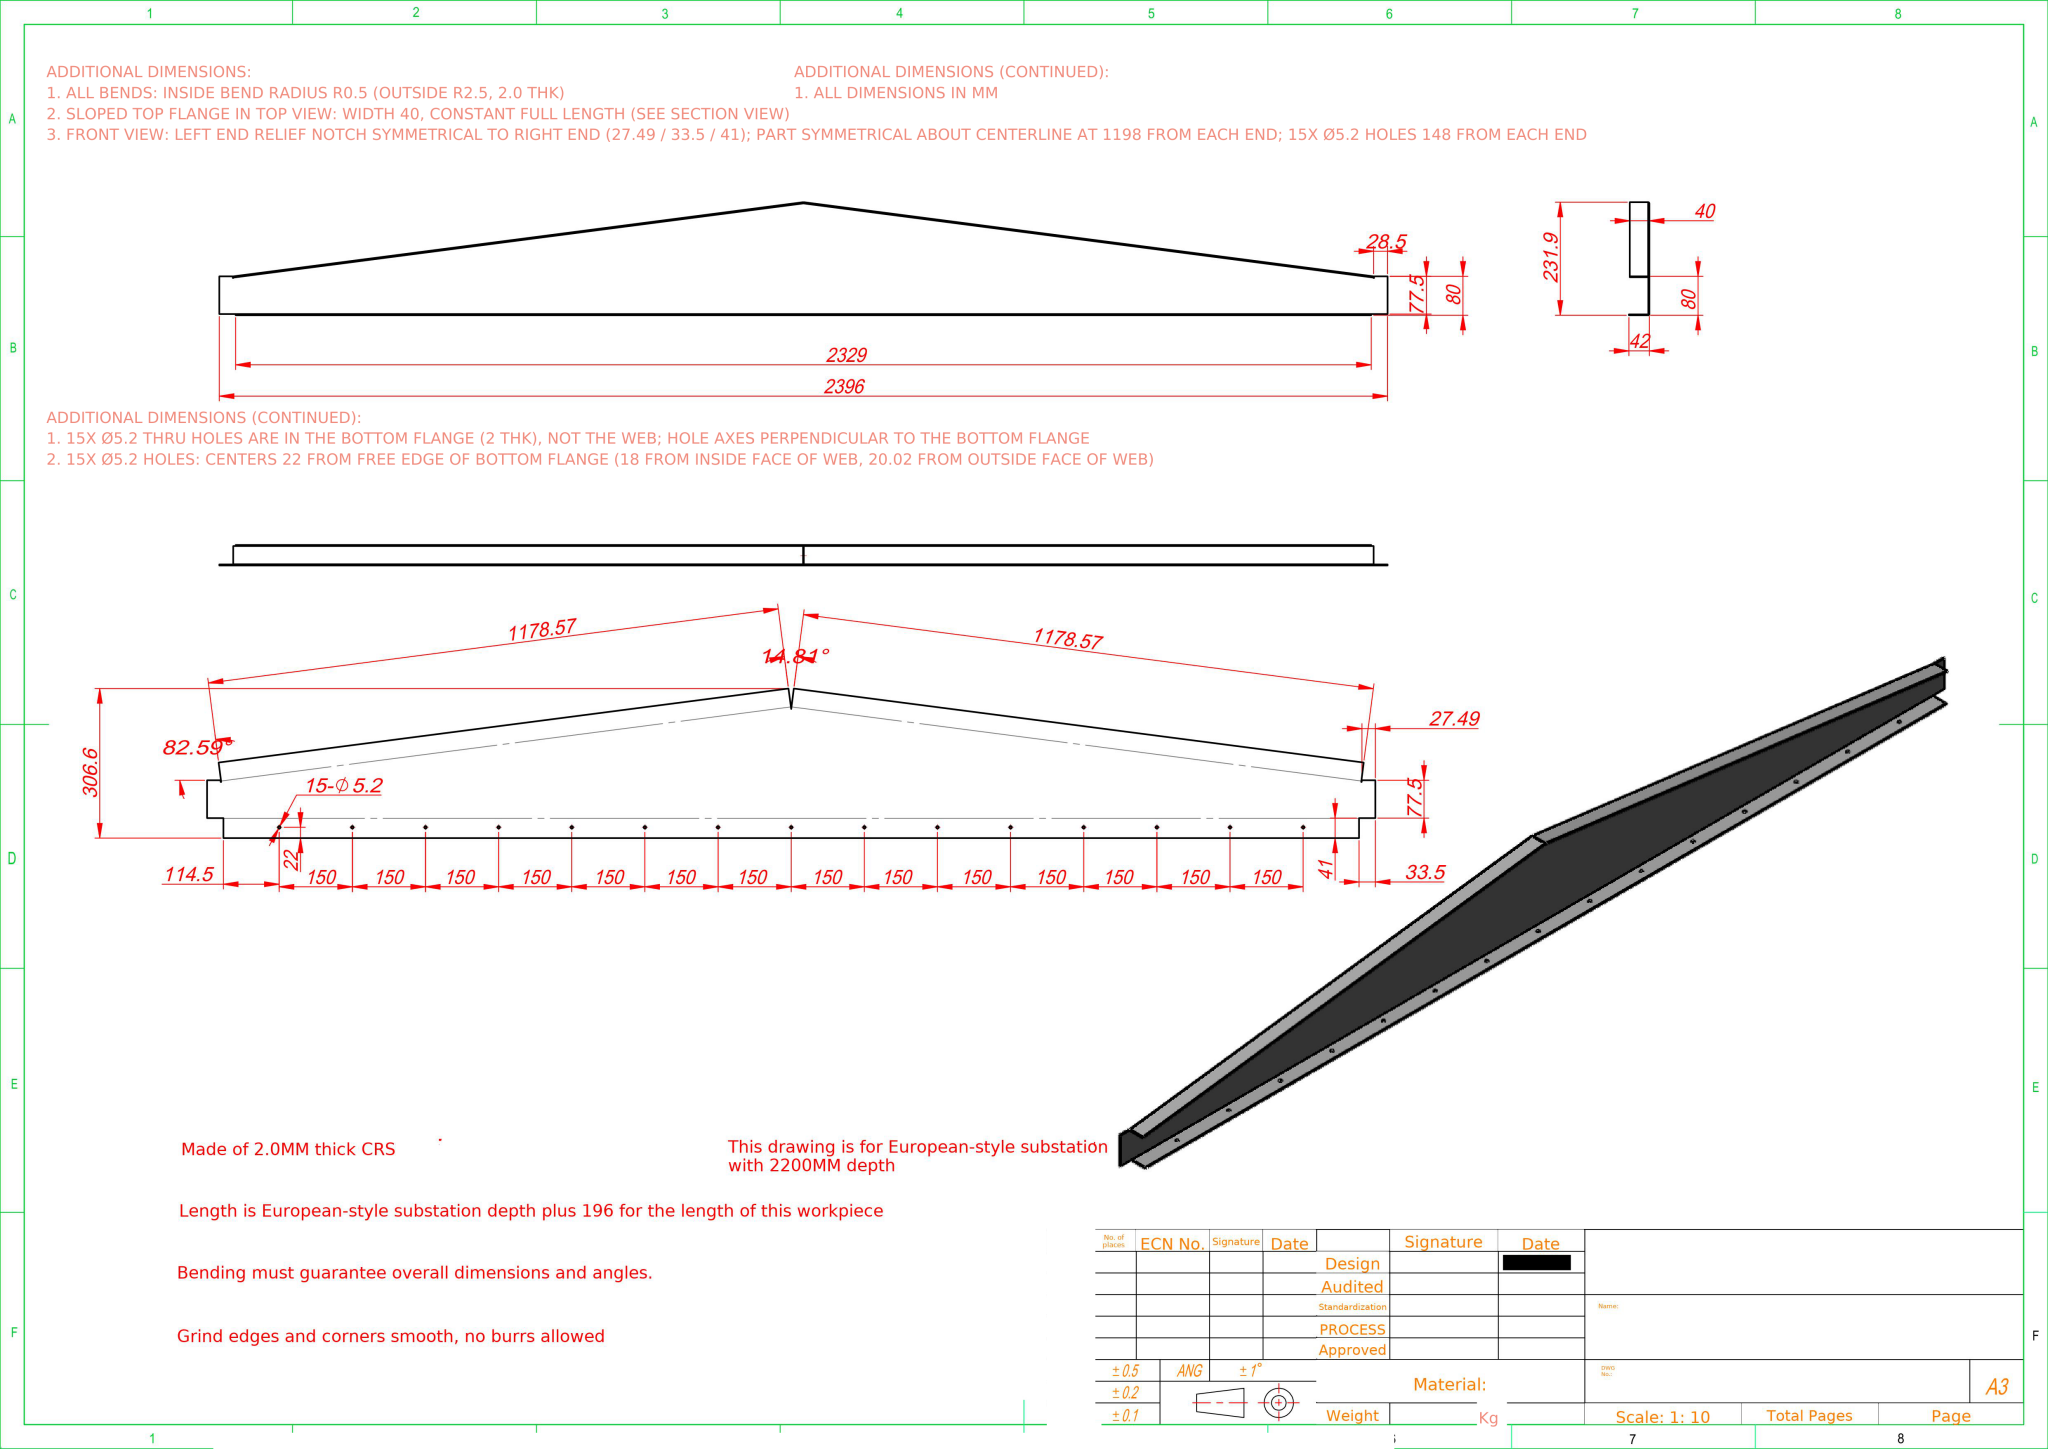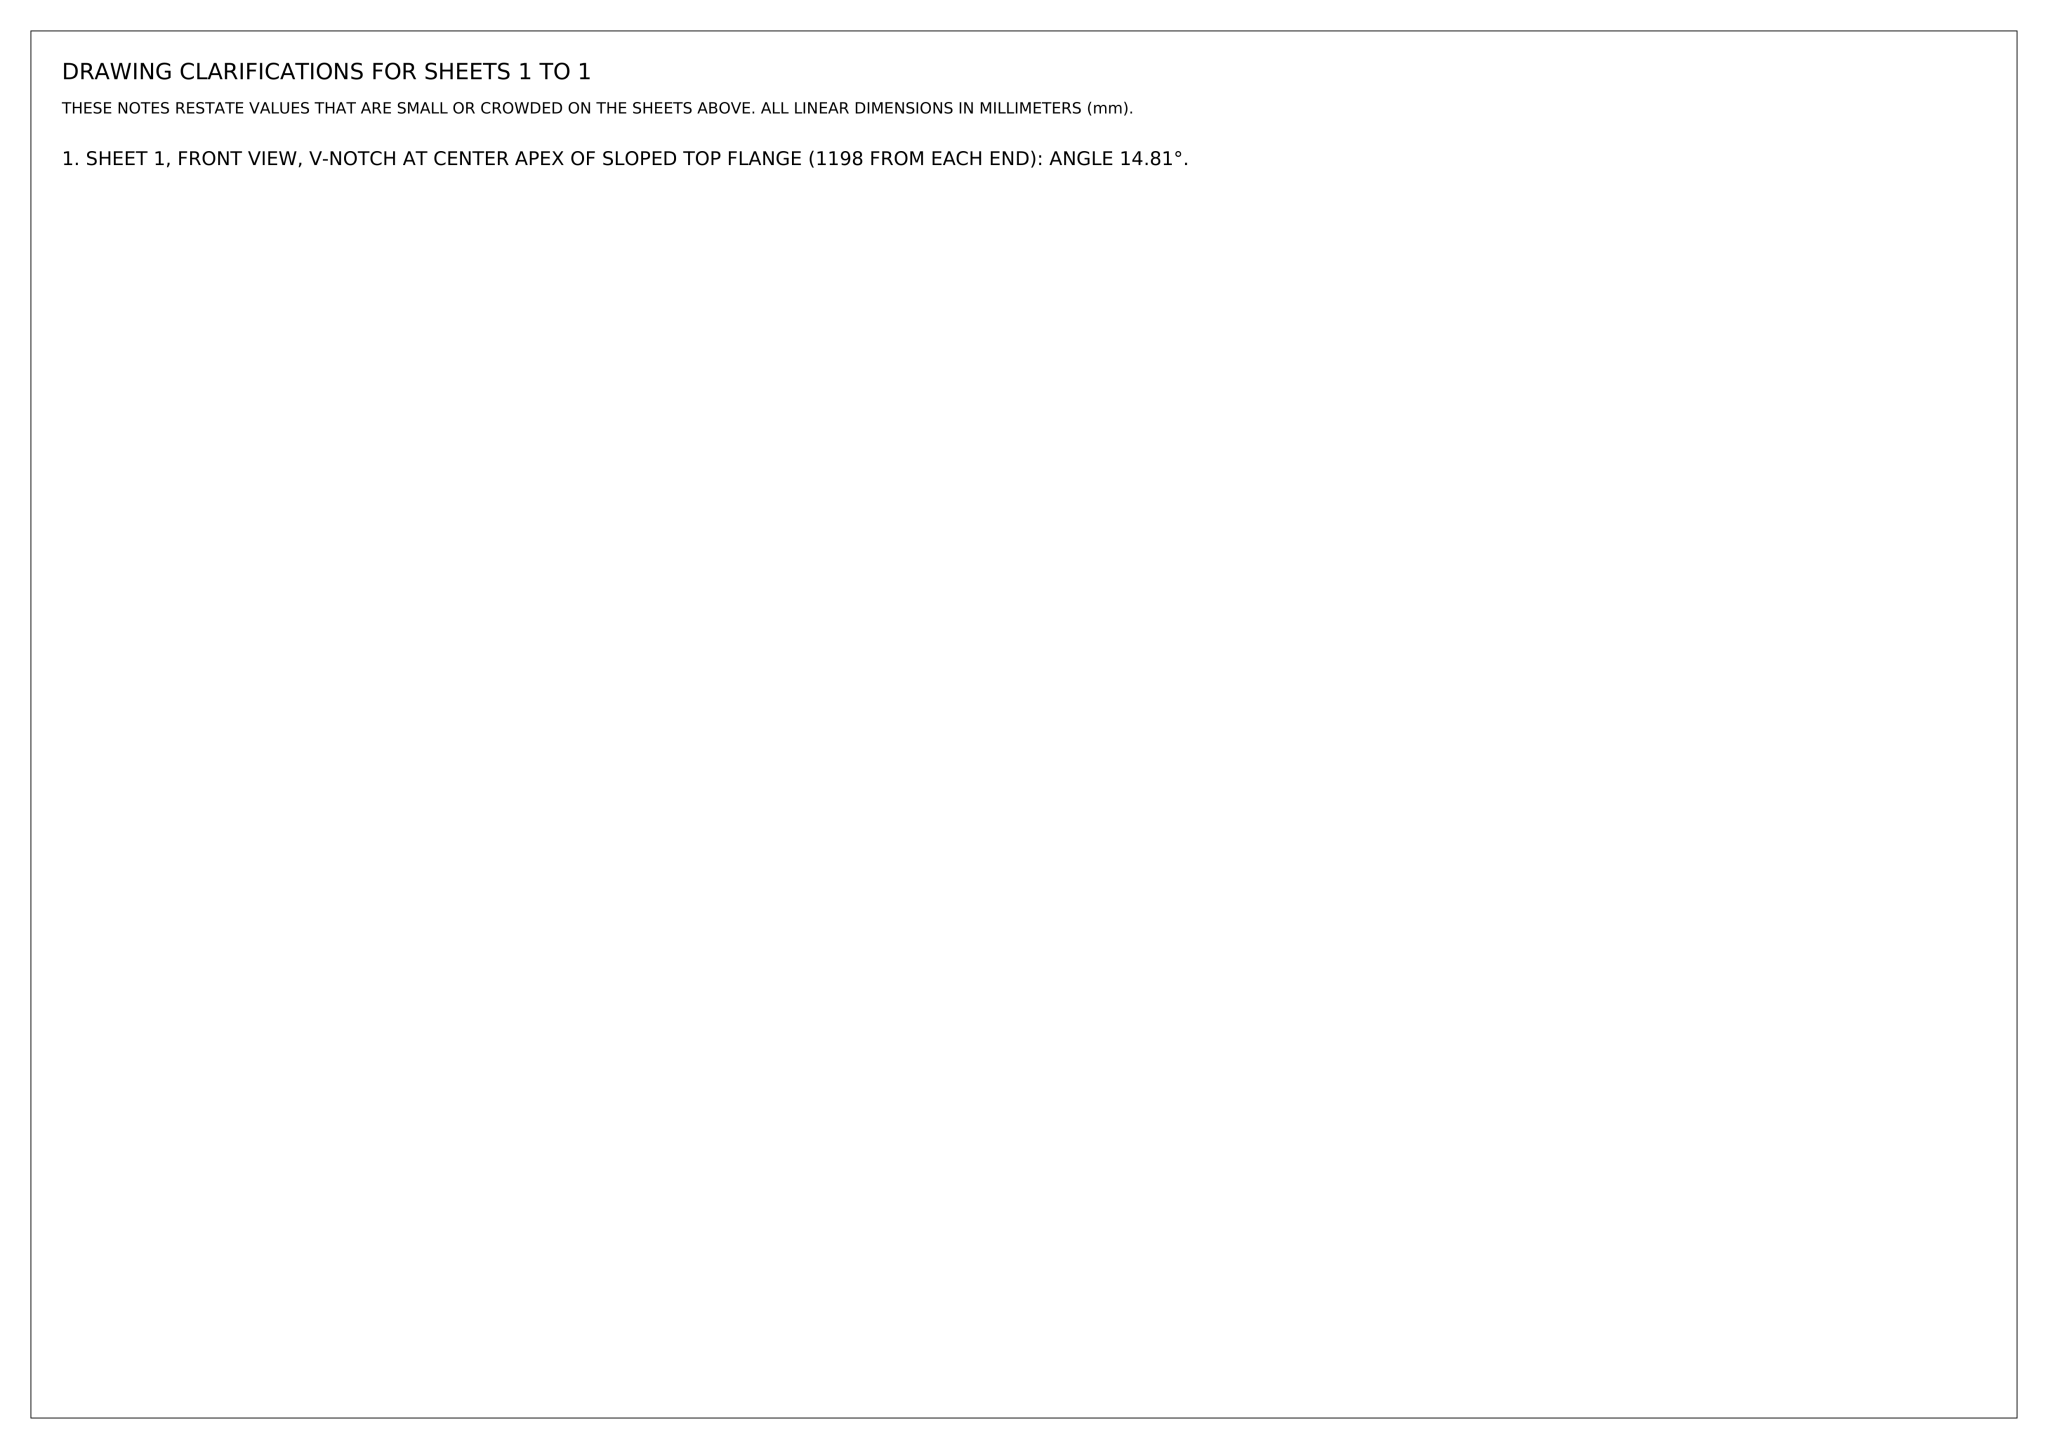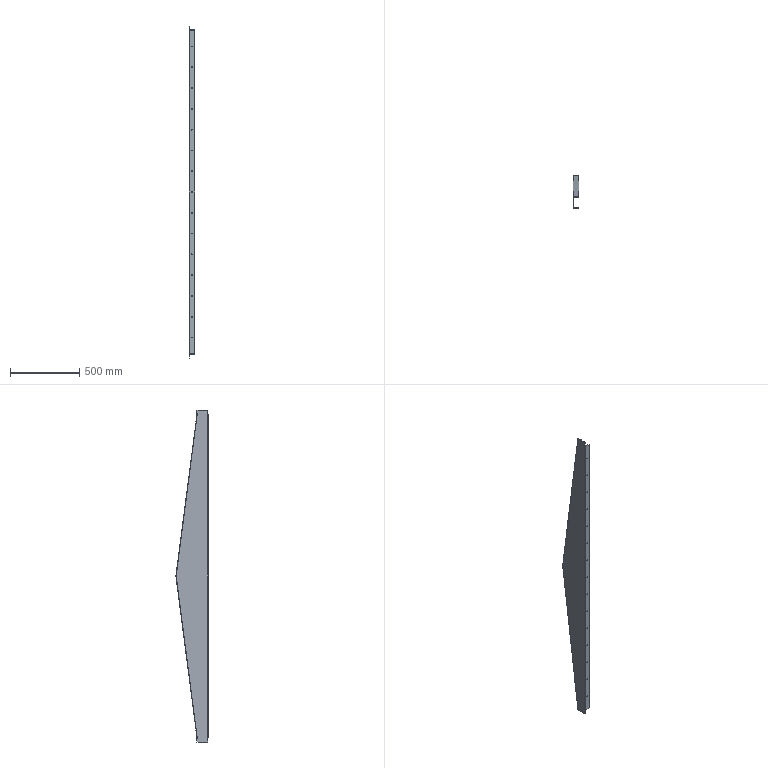Part | NX | mm | 1 solid | 70 faces | box 42 x 231.9 x 2396 mm | volume 1097327 mm3 | cylinder 36 | plane 32 | spline 2 | commonest cylinder face diameters 5.2 x30 5 x3 1 x3